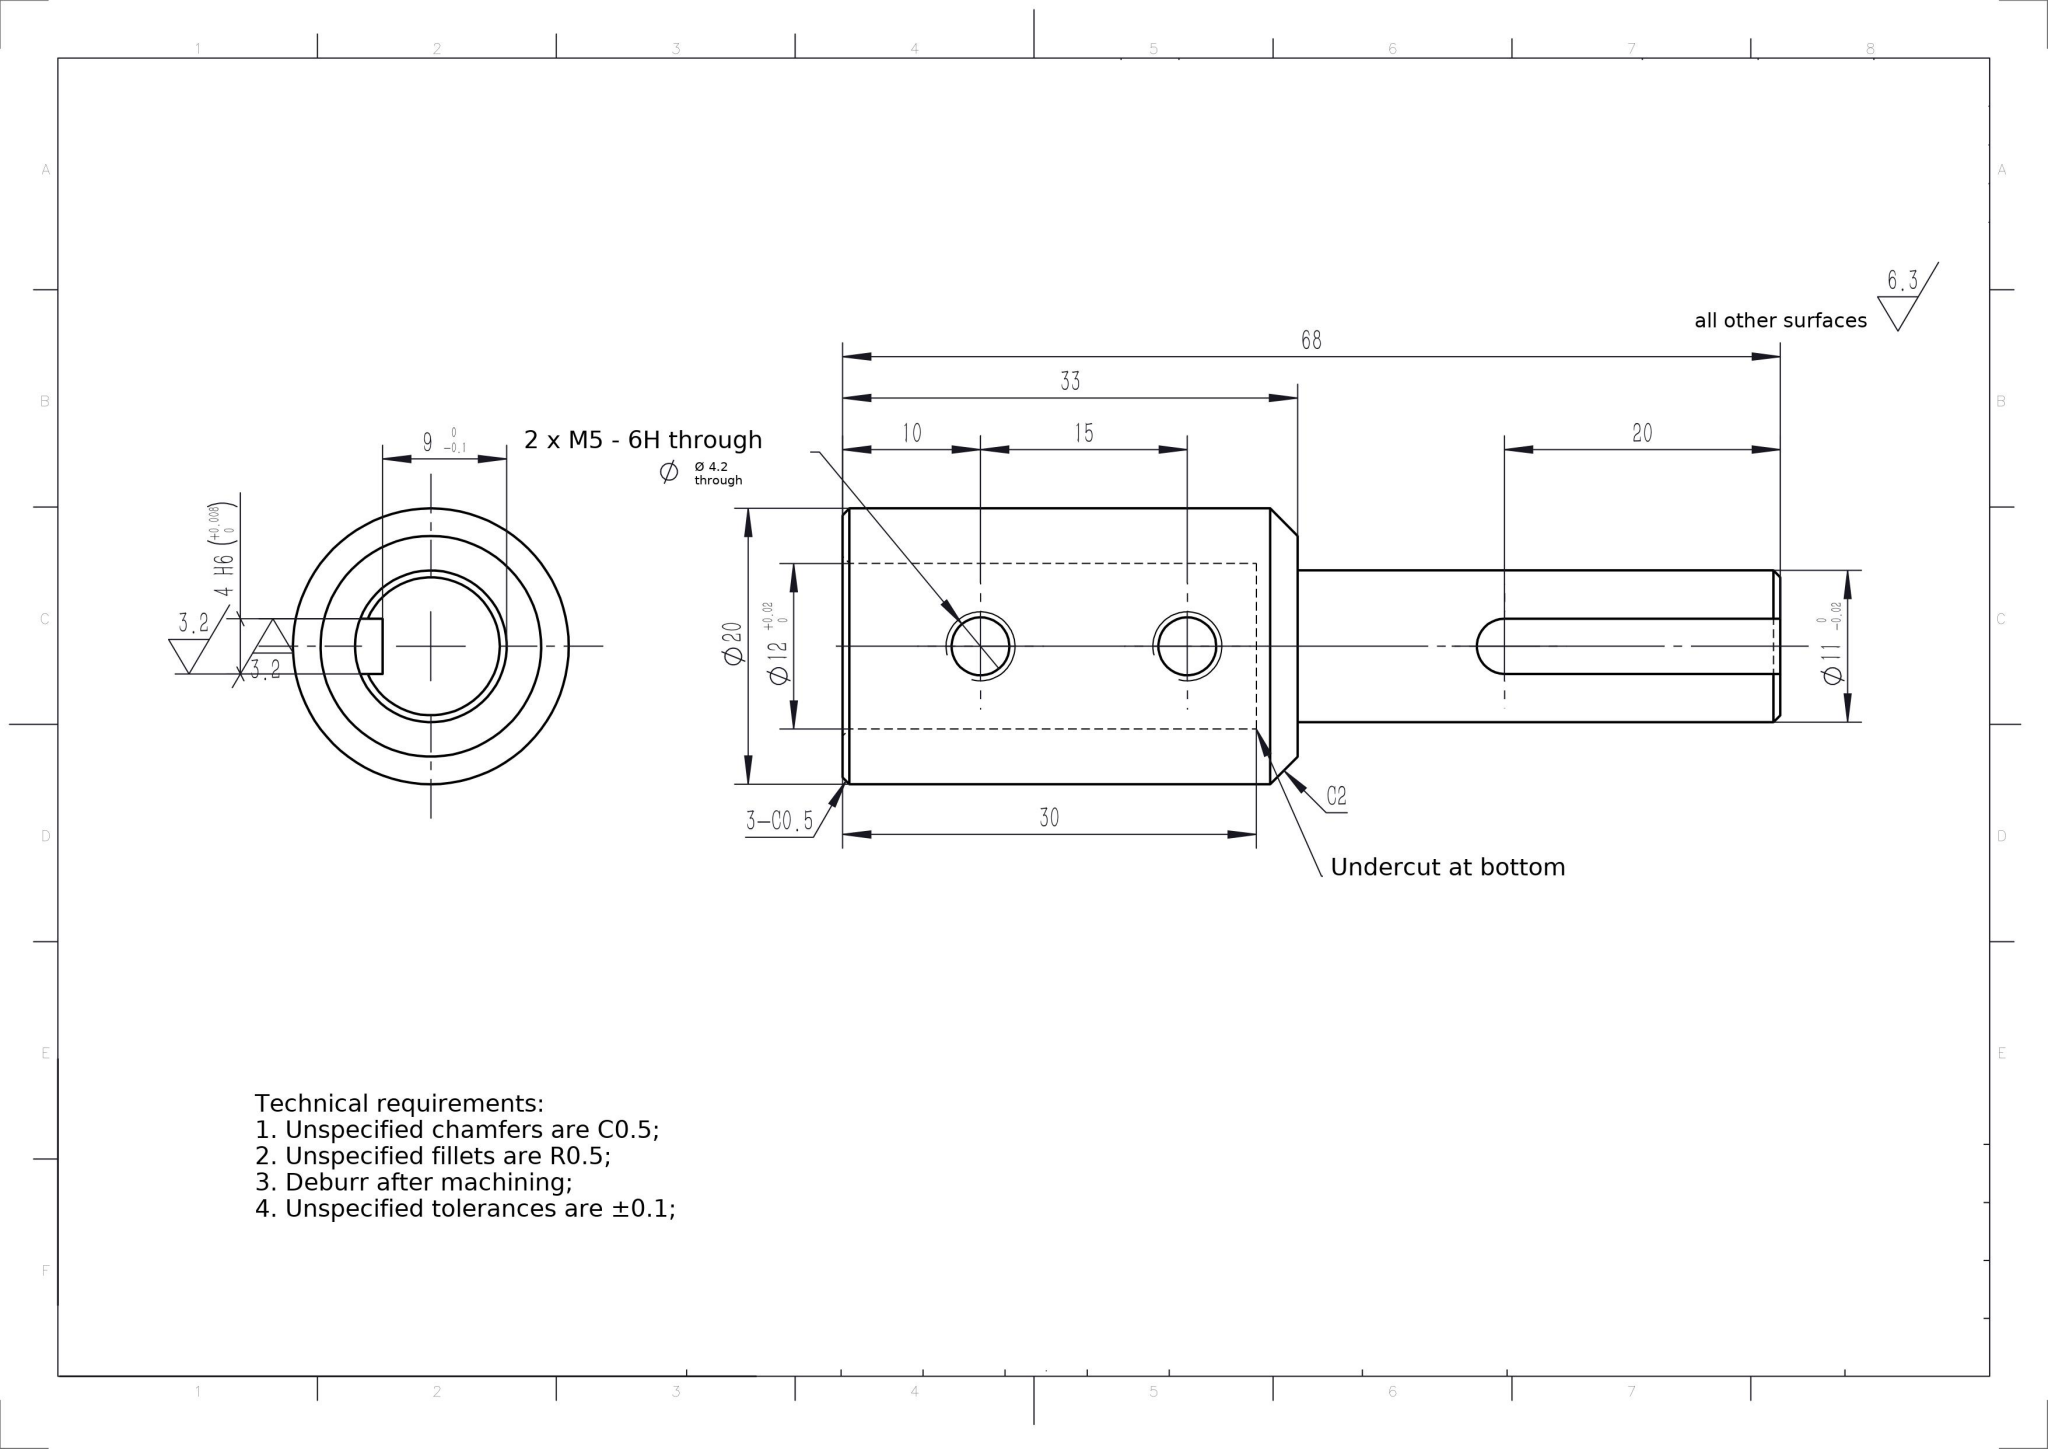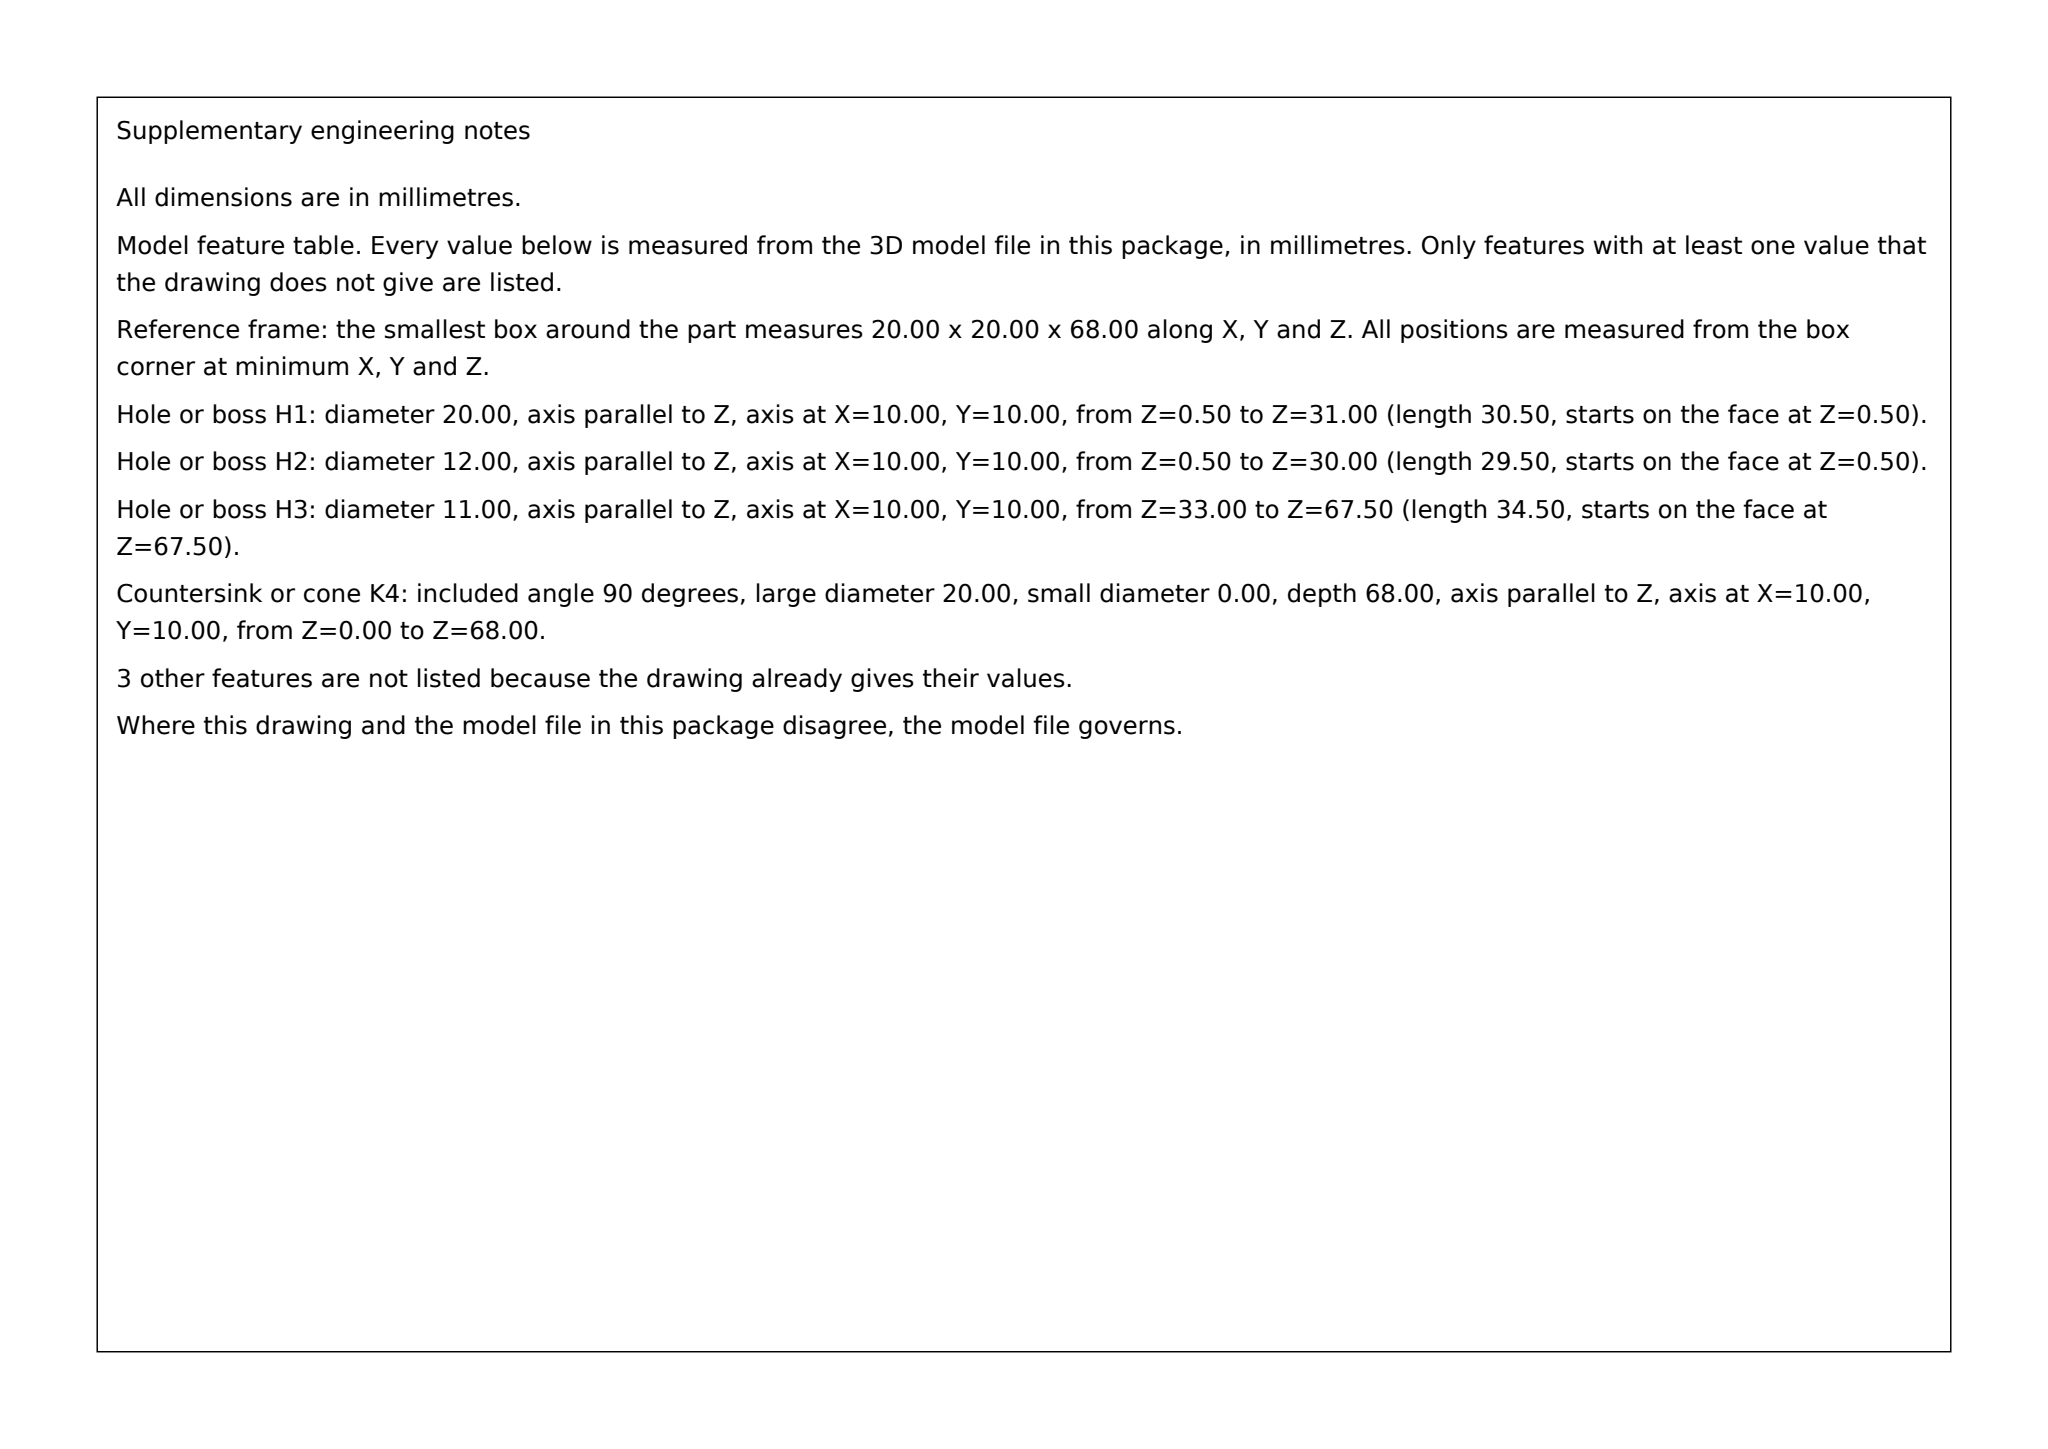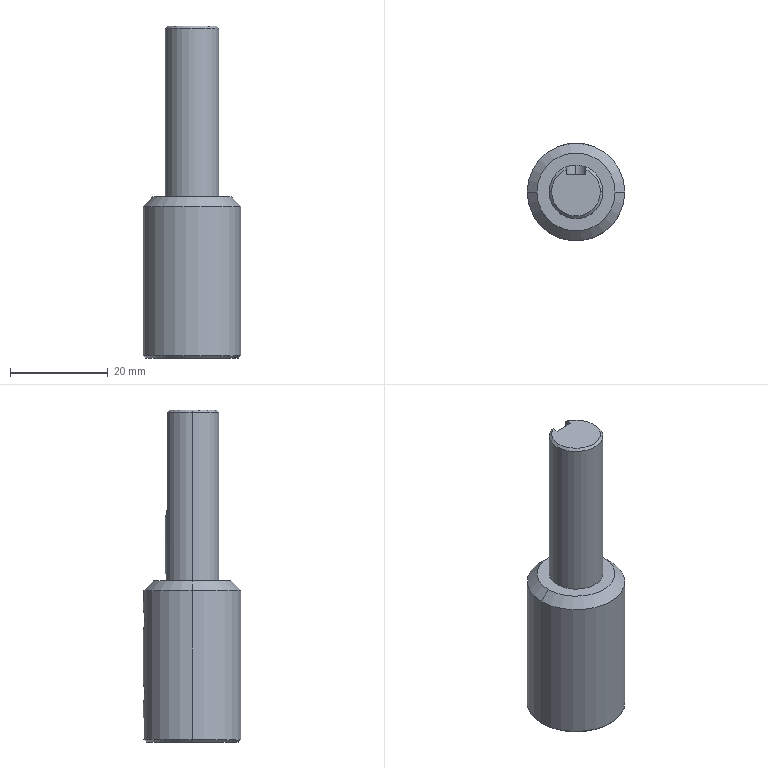Part | SolidWorks | mm | 1 solid | 28 faces | box 20 x 20 x 68 mm | volume 9893 mm3 | cylinder 12 | cone 9 | plane 7 | commonest cylinder face diameters 4.2 x4 4 x2 12 x2 20 x2 11 x2
build123d program:
from build123d import *

# Parameters (mm, degrees)
SKETCH1_R              = 10
BOSS_EXTRUDE1_DEPTH    = 33
SKETCH2_R              = 5.5
BOSS_EXTRUDE2_DEPTH    = 35
SKETCH3_R              = 6
CUT_EXTRUDE1_DEPTH     = 30
M5_TAPPED_HOLE1_REACH  = 50.466
M5_TAPPED_HOLE1_BORE_R = 2.1
CHAMFER1_SIZE          = 2
CUT_EXTRUDE2_START     = 3.5
CUT_EXTRUDE2_DEPTH     = 66.955
CHAMFER2_SIZE          = 0.5


with BuildPart() as part:
    # Sketch1 → Boss-Extrude1 (new body)
    with BuildSketch(Plane.XY):
        Circle(SKETCH1_R)
    extrude(amount=BOSS_EXTRUDE1_DEPTH)

    # Sketch2 → Boss-Extrude2 (add)
    with BuildSketch(Plane.XY.offset(33)):
        Circle(SKETCH2_R)
    extrude(amount=BOSS_EXTRUDE2_DEPTH)

    # Sketch3 → Cut-Extrude1 (cut)
    with BuildSketch(Plane(origin=(0, 0, 0), x_dir=(-1, 0, 0), z_dir=(0, 0, -1))):
        Circle(SKETCH3_R)
    extrude(amount=-CUT_EXTRUDE1_DEPTH, mode=Mode.SUBTRACT)

    # M5 Tapped Hole1 bore (on position points) → M5 Tapped Hole1 (cut, up to next)
    with BuildSketch(Plane(origin=(0, 10, 25), x_dir=(1, 0, 0), z_dir=(0, 1, 0)), mode=Mode.PRIVATE) as m5_tapped_hole1_sk1:
        Circle(M5_TAPPED_HOLE1_BORE_R)
    m5_tapped_hole1_tool1 = extrude(m5_tapped_hole1_sk1.sketch, amount=-M5_TAPPED_HOLE1_REACH, mode=Mode.PRIVATE) & part.part
    # M5 Tapped Hole1 bore (on position points) → M5 Tapped Hole1 (cut, up to next)
    with BuildSketch(Plane(origin=(0, 10, 25), x_dir=(1, 0, 0), z_dir=(0, 1, 0)), mode=Mode.PRIVATE) as m5_tapped_hole1_sk2:
        with Locations((0, 15)):
            Circle(M5_TAPPED_HOLE1_BORE_R)
    m5_tapped_hole1_tool2 = extrude(m5_tapped_hole1_sk2.sketch, amount=-M5_TAPPED_HOLE1_REACH, mode=Mode.PRIVATE) & part.part
    add(m5_tapped_hole1_tool1.solids().sort_by_distance((0, 10, 25))[0], mode=Mode.SUBTRACT)
    add(m5_tapped_hole1_tool2.solids().sort_by_distance((0, 10, 10))[0], mode=Mode.SUBTRACT)

    # Chamfer1
    chamfer1_edges = [part.edges().sort_by_distance(p)[0] for p in [
        (-10, 0, 33),
    ]]
    chamfer(chamfer1_edges, length=CHAMFER1_SIZE)

    # Sketch5 → Cut-Extrude2 (cut, through all)
    with BuildSketch(Plane(origin=(0, 0, 0), x_dir=(1, 0, 0), z_dir=(0, 1, 0)).offset(CUT_EXTRUDE2_START)):
        with BuildLine():
            Line((-2, -68), (-2, -48))
            ThreePointArc((-2, -48), (0, -46), (2, -48))
            Line((2, -48), (2, -68))
            ThreePointArc((2, -68), (0, -70), (-2, -68))
        make_face()
    extrude(amount=CUT_EXTRUDE2_DEPTH, mode=Mode.SUBTRACT)

    # Chamfer2
    chamfer2_edges = [part.edges().sort_by_distance(p)[0] for p in [
        (6, 0, 0),
        (-10, 0, 0),
        (-3.102, -4.541, 68),
    ]]
    chamfer(chamfer2_edges, length=CHAMFER2_SIZE)


solid = part.part